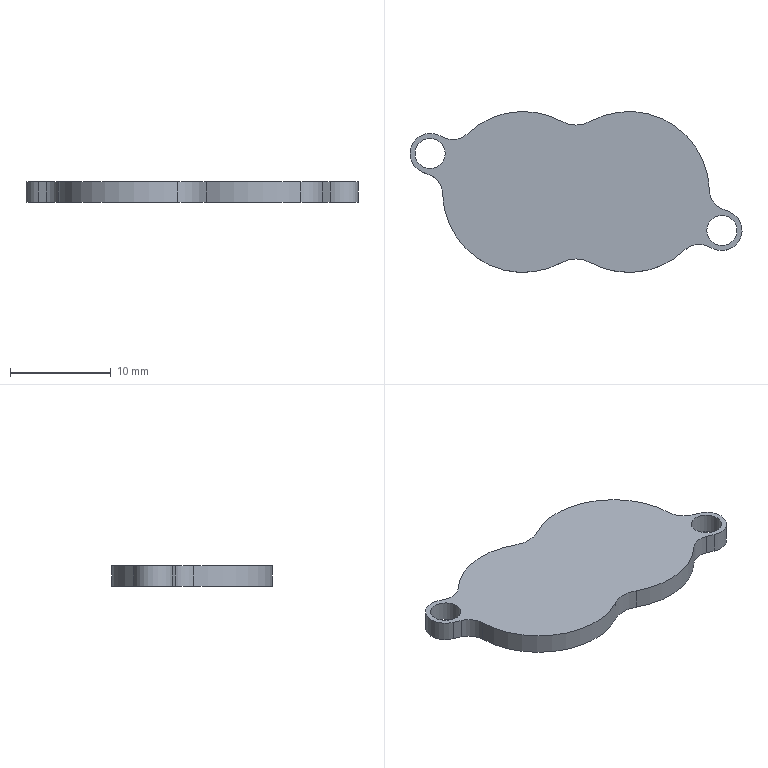Component | NX | SMALL_COVER | 1 solid | 20 faces | volume 748 mm3 | cylinder 14 | plane 6 | commonest cylinder face diameters 4 x6 16 x4 6 x2 3 x2